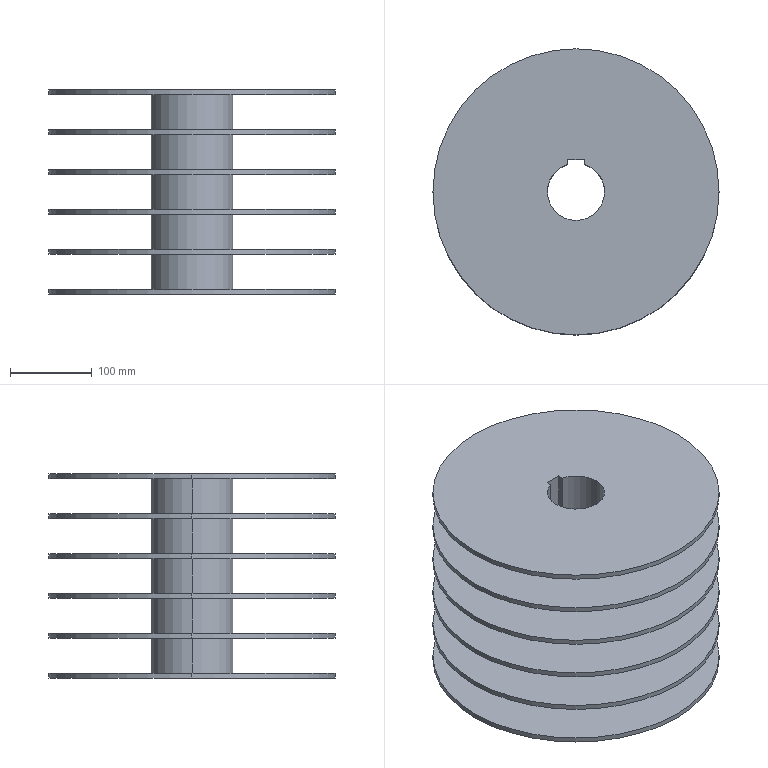Component | SolidWorks | HammerPiece-1_ToolHolder-1 | 1 solid | 40 faces | box 350 x 350 x 250 mm | volume 4155334 mm3 | cylinder 25 | plane 15 | commonest cylinder face diameters 350 x12 100 x10 70 x3
STEP:
#1=CARTESIAN_POINT('',(6.89,8.839,-4.921));
#2=VERTEX_POINT('',#1);
#3=CARTESIAN_POINT('',(9.646,8.839,-4.921));
#4=VERTEX_POINT('',#3);
#5=CARTESIAN_POINT('',(8.268,8.839,-4.921));
#6=DIRECTION('',(0.,0.,1.));
#7=DIRECTION('',(1.,0.,0.));
#8=AXIS2_PLACEMENT_3D('',#5,#6,#7);
#9=CIRCLE('',#8,1.378);
#10=EDGE_CURVE('',#2,#4,#9,.T.);
#11=ORIENTED_EDGE('',*,*,#10,.F.);
#12=CARTESIAN_POINT('',(6.89,8.839,4.921));
#13=VERTEX_POINT('',#12);
#14=CARTESIAN_POINT('',(6.89,8.839,-0.));
#15=DIRECTION('',(0.,0.,1.));
#16=VECTOR('',#15,39.37);
#17=LINE('',#14,#16);
#18=EDGE_CURVE('',#2,#13,#17,.T.);
#19=ORIENTED_EDGE('',*,*,#18,.T.);
#20=CARTESIAN_POINT('',(9.646,8.839,4.921));
#21=VERTEX_POINT('',#20);
#22=CARTESIAN_POINT('',(8.268,8.839,4.921));
#23=DIRECTION('',(0.,0.,1.));
#24=DIRECTION('',(1.,0.,0.));
#25=AXIS2_PLACEMENT_3D('',#22,#23,#24);
#26=CIRCLE('',#25,1.378);
#27=EDGE_CURVE('',#13,#21,#26,.T.);
#28=ORIENTED_EDGE('',*,*,#27,.T.);
#29=CARTESIAN_POINT('',(9.646,8.839,-0.));
#30=DIRECTION('',(0.,0.,1.));
#31=VECTOR('',#30,39.37);
#32=LINE('',#29,#31);
#33=EDGE_CURVE('',#4,#21,#32,.T.);
#34=ORIENTED_EDGE('',*,*,#33,.F.);
#35=EDGE_LOOP('',(#11,#19,#28,#34));
#36=FACE_OUTER_BOUND('',#35,.T.);
#37=CARTESIAN_POINT('',(8.268,8.839,-0.));
#38=DIRECTION('',(0.,0.,1.));
#39=DIRECTION('',(1.,0.,0.));
#40=AXIS2_PLACEMENT_3D('',#37,#38,#39);
#41=CYLINDRICAL_SURFACE('',#40,1.378);
#42=ADVANCED_FACE('',(#36),#41,.F.);
#43=CARTESIAN_POINT('',(8.661,10.159,-4.921));
#44=VERTEX_POINT('',#43);
#45=CARTESIAN_POINT('',(8.268,8.839,-4.921));
#46=DIRECTION('',(0.,0.,1.));
#47=DIRECTION('',(1.,0.,0.));
#48=AXIS2_PLACEMENT_3D('',#45,#46,#47);
#49=CIRCLE('',#48,1.378);
#50=EDGE_CURVE('',#4,#44,#49,.T.);
#51=ORIENTED_EDGE('',*,*,#50,.F.);
#52=ORIENTED_EDGE('',*,*,#33,.T.);
#53=CARTESIAN_POINT('',(8.661,10.159,4.921));
#54=VERTEX_POINT('',#53);
#55=CARTESIAN_POINT('',(8.268,8.839,4.921));
#56=DIRECTION('',(0.,0.,1.));
#57=DIRECTION('',(1.,0.,0.));
#58=AXIS2_PLACEMENT_3D('',#55,#56,#57);
#59=CIRCLE('',#58,1.378);
#60=EDGE_CURVE('',#21,#54,#59,.T.);
#61=ORIENTED_EDGE('',*,*,#60,.T.);
#62=CARTESIAN_POINT('',(8.661,10.159,5.157));
#63=DIRECTION('',(0.,0.,-1.));
#64=VECTOR('',#63,39.37);
#65=LINE('',#62,#64);
#66=EDGE_CURVE('',#54,#44,#65,.T.);
#67=ORIENTED_EDGE('',*,*,#66,.T.);
#68=EDGE_LOOP('',(#51,#52,#61,#67));
#69=FACE_OUTER_BOUND('',#68,.T.);
#70=CARTESIAN_POINT('',(8.268,8.839,-0.));
#71=DIRECTION('',(0.,0.,1.));
#72=DIRECTION('',(1.,0.,0.));
#73=AXIS2_PLACEMENT_3D('',#70,#71,#72);
#74=CYLINDRICAL_SURFACE('',#73,1.378);
#75=ADVANCED_FACE('',(#69),#74,.F.);
#76=CARTESIAN_POINT('',(15.157,8.839,4.685));
#77=VERTEX_POINT('',#76);
#78=CARTESIAN_POINT('',(1.378,8.839,4.685));
#79=VERTEX_POINT('',#78);
#80=CARTESIAN_POINT('',(8.268,8.839,4.685));
#81=DIRECTION('',(0.,0.,1.));
#82=DIRECTION('',(1.,0.,0.));
#83=AXIS2_PLACEMENT_3D('',#80,#81,#82);
#84=CIRCLE('',#83,6.89);
#85=EDGE_CURVE('',#77,#79,#84,.T.);
#86=ORIENTED_EDGE('',*,*,#85,.T.);
#87=CARTESIAN_POINT('',(1.378,8.839,4.921));
#88=VERTEX_POINT('',#87);
#89=CARTESIAN_POINT('',(1.378,8.839,-0.));
#90=DIRECTION('',(0.,0.,1.));
#91=VECTOR('',#90,39.37);
#92=LINE('',#89,#91);
#93=EDGE_CURVE('',#79,#88,#92,.T.);
#94=ORIENTED_EDGE('',*,*,#93,.T.);
#95=CARTESIAN_POINT('',(15.157,8.839,4.921));
#96=VERTEX_POINT('',#95);
#97=CARTESIAN_POINT('',(8.268,8.839,4.921));
#98=DIRECTION('',(0.,0.,-1.));
#99=DIRECTION('',(1.,0.,0.));
#100=AXIS2_PLACEMENT_3D('',#97,#98,#99);
#101=CIRCLE('',#100,6.89);
#102=EDGE_CURVE('',#88,#96,#101,.T.);
#103=ORIENTED_EDGE('',*,*,#102,.T.);
#104=CARTESIAN_POINT('',(15.157,8.839,-0.));
#105=DIRECTION('',(0.,0.,1.));
#106=VECTOR('',#105,39.37);
#107=LINE('',#104,#106);
#108=EDGE_CURVE('',#77,#96,#107,.T.);
#109=ORIENTED_EDGE('',*,*,#108,.F.);
#110=EDGE_LOOP('',(#86,#94,#103,#109));
#111=FACE_OUTER_BOUND('',#110,.T.);
#112=CARTESIAN_POINT('',(8.268,8.839,-0.));
#113=DIRECTION('',(0.,0.,1.));
#114=DIRECTION('',(1.,0.,0.));
#115=AXIS2_PLACEMENT_3D('',#112,#113,#114);
#116=CYLINDRICAL_SURFACE('',#115,6.89);
#117=ADVANCED_FACE('',(#111),#116,.T.);
#118=CARTESIAN_POINT('',(15.157,8.839,-4.921));
#119=VERTEX_POINT('',#118);
#120=CARTESIAN_POINT('',(1.378,8.839,-4.921));
#121=VERTEX_POINT('',#120);
#122=CARTESIAN_POINT('',(8.268,8.839,-4.921));
#123=DIRECTION('',(0.,0.,1.));
#124=DIRECTION('',(1.,0.,0.));
#125=AXIS2_PLACEMENT_3D('',#122,#123,#124);
#126=CIRCLE('',#125,6.89);
#127=EDGE_CURVE('',#119,#121,#126,.T.);
#128=ORIENTED_EDGE('',*,*,#127,.T.);
#129=CARTESIAN_POINT('',(1.378,8.839,-4.685));
#130=VERTEX_POINT('',#129);
#131=CARTESIAN_POINT('',(1.378,8.839,-0.));
#132=DIRECTION('',(0.,0.,1.));
#133=VECTOR('',#132,39.37);
#134=LINE('',#131,#133);
#135=EDGE_CURVE('',#121,#130,#134,.T.);
#136=ORIENTED_EDGE('',*,*,#135,.T.);
#137=CARTESIAN_POINT('',(15.157,8.839,-4.685));
#138=VERTEX_POINT('',#137);
#139=CARTESIAN_POINT('',(8.268,8.839,-4.685));
#140=DIRECTION('',(0.,0.,-1.));
#141=DIRECTION('',(1.,0.,0.));
#142=AXIS2_PLACEMENT_3D('',#139,#140,#141);
#143=CIRCLE('',#142,6.89);
#144=EDGE_CURVE('',#130,#138,#143,.T.);
#145=ORIENTED_EDGE('',*,*,#144,.T.);
#146=CARTESIAN_POINT('',(15.157,8.839,-0.));
#147=DIRECTION('',(0.,0.,1.));
#148=VECTOR('',#147,39.37);
#149=LINE('',#146,#148);
#150=EDGE_CURVE('',#119,#138,#149,.T.);
#151=ORIENTED_EDGE('',*,*,#150,.F.);
#152=EDGE_LOOP('',(#128,#136,#145,#151));
#153=FACE_OUTER_BOUND('',#152,.T.);
#154=CARTESIAN_POINT('',(8.268,8.839,-0.));
#155=DIRECTION('',(0.,0.,1.));
#156=DIRECTION('',(1.,0.,0.));
#157=AXIS2_PLACEMENT_3D('',#154,#155,#156);
#158=CYLINDRICAL_SURFACE('',#157,6.89);
#159=ADVANCED_FACE('',(#153),#158,.T.);
#160=CARTESIAN_POINT('',(10.236,8.839,3.));
#161=VERTEX_POINT('',#160);
#162=CARTESIAN_POINT('',(6.299,8.839,3.));
#163=VERTEX_POINT('',#162);
#164=CARTESIAN_POINT('',(8.268,8.839,3.));
#165=DIRECTION('',(0.,0.,1.));
#166=DIRECTION('',(1.,0.,0.));
#167=AXIS2_PLACEMENT_3D('',#164,#165,#166);
#168=CIRCLE('',#167,1.969);
#169=EDGE_CURVE('',#161,#163,#168,.T.);
#170=ORIENTED_EDGE('',*,*,#169,.T.);
#171=CARTESIAN_POINT('',(6.299,8.839,4.685));
#172=VERTEX_POINT('',#171);
#173=CARTESIAN_POINT('',(6.299,8.839,-10.489));
#174=DIRECTION('',(0.,0.,1.));
#175=VECTOR('',#174,39.37);
#176=LINE('',#173,#175);
#177=EDGE_CURVE('',#163,#172,#176,.T.);
#178=ORIENTED_EDGE('',*,*,#177,.T.);
#179=CARTESIAN_POINT('',(10.236,8.839,4.685));
#180=VERTEX_POINT('',#179);
#181=CARTESIAN_POINT('',(8.268,8.839,4.685));
#182=DIRECTION('',(0.,0.,-1.));
#183=DIRECTION('',(1.,0.,0.));
#184=AXIS2_PLACEMENT_3D('',#181,#182,#183);
#185=CIRCLE('',#184,1.969);
#186=EDGE_CURVE('',#172,#180,#185,.T.);
#187=ORIENTED_EDGE('',*,*,#186,.T.);
#188=CARTESIAN_POINT('',(10.236,8.839,-10.489));
#189=DIRECTION('',(0.,0.,1.));
#190=VECTOR('',#189,39.37);
#191=LINE('',#188,#190);
#192=EDGE_CURVE('',#161,#180,#191,.T.);
#193=ORIENTED_EDGE('',*,*,#192,.F.);
#194=EDGE_LOOP('',(#170,#178,#187,#193));
#195=FACE_OUTER_BOUND('',#194,.T.);
#196=CARTESIAN_POINT('',(8.268,8.839,-10.489));
#197=DIRECTION('',(0.,0.,1.));
#198=DIRECTION('',(1.,0.,0.));
#199=AXIS2_PLACEMENT_3D('',#196,#197,#198);
#200=CYLINDRICAL_SURFACE('',#199,1.969);
#201=ADVANCED_FACE('',(#195),#200,.T.);
#202=CARTESIAN_POINT('',(10.236,8.839,-4.685));
#203=VERTEX_POINT('',#202);
#204=CARTESIAN_POINT('',(6.299,8.839,-4.685));
#205=VERTEX_POINT('',#204);
#206=CARTESIAN_POINT('',(8.268,8.839,-4.685));
#207=DIRECTION('',(0.,0.,1.));
#208=DIRECTION('',(1.,0.,0.));
#209=AXIS2_PLACEMENT_3D('',#206,#207,#208);
#210=CIRCLE('',#209,1.969);
#211=EDGE_CURVE('',#203,#205,#210,.T.);
#212=ORIENTED_EDGE('',*,*,#211,.T.);
#213=CARTESIAN_POINT('',(6.299,8.839,-3.));
#214=VERTEX_POINT('',#213);
#215=CARTESIAN_POINT('',(6.299,8.839,-10.489));
#216=DIRECTION('',(0.,0.,1.));
#217=VECTOR('',#216,39.37);
#218=LINE('',#215,#217);
#219=EDGE_CURVE('',#205,#214,#218,.T.);
#220=ORIENTED_EDGE('',*,*,#219,.T.);
#221=CARTESIAN_POINT('',(10.236,8.839,-3.));
#222=VERTEX_POINT('',#221);
#223=CARTESIAN_POINT('',(8.268,8.839,-3.));
#224=DIRECTION('',(0.,0.,-1.));
#225=DIRECTION('',(1.,0.,0.));
#226=AXIS2_PLACEMENT_3D('',#223,#224,#225);
#227=CIRCLE('',#226,1.969);
#228=EDGE_CURVE('',#214,#222,#227,.T.);
#229=ORIENTED_EDGE('',*,*,#228,.T.);
#230=CARTESIAN_POINT('',(10.236,8.839,-10.489));
#231=DIRECTION('',(0.,0.,1.));
#232=VECTOR('',#231,39.37);
#233=LINE('',#230,#232);
#234=EDGE_CURVE('',#203,#222,#233,.T.);
#235=ORIENTED_EDGE('',*,*,#234,.F.);
#236=EDGE_LOOP('',(#212,#220,#229,#235));
#237=FACE_OUTER_BOUND('',#236,.T.);
#238=CARTESIAN_POINT('',(8.268,8.839,-10.489));
#239=DIRECTION('',(0.,0.,1.));
#240=DIRECTION('',(1.,0.,0.));
#241=AXIS2_PLACEMENT_3D('',#238,#239,#240);
#242=CYLINDRICAL_SURFACE('',#241,1.969);
#243=ADVANCED_FACE('',(#237),#242,.T.);
#244=CARTESIAN_POINT('',(15.157,8.839,2.764));
#245=VERTEX_POINT('',#244);
#246=CARTESIAN_POINT('',(1.378,8.839,2.764));
#247=VERTEX_POINT('',#246);
#248=CARTESIAN_POINT('',(8.268,8.839,2.764));
#249=DIRECTION('',(0.,0.,1.));
#250=DIRECTION('',(1.,0.,0.));
#251=AXIS2_PLACEMENT_3D('',#248,#249,#250);
#252=CIRCLE('',#251,6.89);
#253=EDGE_CURVE('',#245,#247,#252,.T.);
#254=ORIENTED_EDGE('',*,*,#253,.T.);
#255=CARTESIAN_POINT('',(1.378,8.839,3.));
#256=VERTEX_POINT('',#255);
#257=CARTESIAN_POINT('',(1.378,8.839,-0.));
#258=DIRECTION('',(0.,0.,1.));
#259=VECTOR('',#258,39.37);
#260=LINE('',#257,#259);
#261=EDGE_CURVE('',#247,#256,#260,.T.);
#262=ORIENTED_EDGE('',*,*,#261,.T.);
#263=CARTESIAN_POINT('',(15.157,8.839,3.));
#264=VERTEX_POINT('',#263);
#265=CARTESIAN_POINT('',(8.268,8.839,3.));
#266=DIRECTION('',(0.,0.,-1.));
#267=DIRECTION('',(1.,0.,0.));
#268=AXIS2_PLACEMENT_3D('',#265,#266,#267);
#269=CIRCLE('',#268,6.89);
#270=EDGE_CURVE('',#256,#264,#269,.T.);
#271=ORIENTED_EDGE('',*,*,#270,.T.);
#272=CARTESIAN_POINT('',(15.157,8.839,-0.));
#273=DIRECTION('',(0.,0.,1.));
#274=VECTOR('',#273,39.37);
#275=LINE('',#272,#274);
#276=EDGE_CURVE('',#245,#264,#275,.T.);
#277=ORIENTED_EDGE('',*,*,#276,.F.);
#278=EDGE_LOOP('',(#254,#262,#271,#277));
#279=FACE_OUTER_BOUND('',#278,.T.);
#280=CARTESIAN_POINT('',(8.268,8.839,-0.));
#281=DIRECTION('',(0.,0.,1.));
#282=DIRECTION('',(1.,0.,0.));
#283=AXIS2_PLACEMENT_3D('',#280,#281,#282);
#284=CYLINDRICAL_SURFACE('',#283,6.89);
#285=ADVANCED_FACE('',(#279),#284,.T.);
#286=CARTESIAN_POINT('',(15.157,8.839,-3.));
#287=VERTEX_POINT('',#286);
#288=CARTESIAN_POINT('',(1.378,8.839,-3.));
#289=VERTEX_POINT('',#288);
#290=CARTESIAN_POINT('',(8.268,8.839,-3.));
#291=DIRECTION('',(0.,0.,1.));
#292=DIRECTION('',(1.,0.,0.));
#293=AXIS2_PLACEMENT_3D('',#290,#291,#292);
#294=CIRCLE('',#293,6.89);
#295=EDGE_CURVE('',#287,#289,#294,.T.);
#296=ORIENTED_EDGE('',*,*,#295,.T.);
#297=CARTESIAN_POINT('',(1.378,8.839,-2.764));
#298=VERTEX_POINT('',#297);
#299=CARTESIAN_POINT('',(1.378,8.839,-0.));
#300=DIRECTION('',(0.,0.,1.));
#301=VECTOR('',#300,39.37);
#302=LINE('',#299,#301);
#303=EDGE_CURVE('',#289,#298,#302,.T.);
#304=ORIENTED_EDGE('',*,*,#303,.T.);
#305=CARTESIAN_POINT('',(15.157,8.839,-2.764));
#306=VERTEX_POINT('',#305);
#307=CARTESIAN_POINT('',(8.268,8.839,-2.764));
#308=DIRECTION('',(0.,0.,-1.));
#309=DIRECTION('',(1.,0.,0.));
#310=AXIS2_PLACEMENT_3D('',#307,#308,#309);
#311=CIRCLE('',#310,6.89);
#312=EDGE_CURVE('',#298,#306,#311,.T.);
#313=ORIENTED_EDGE('',*,*,#312,.T.);
#314=CARTESIAN_POINT('',(15.157,8.839,-0.));
#315=DIRECTION('',(0.,0.,1.));
#316=VECTOR('',#315,39.37);
#317=LINE('',#314,#316);
#318=EDGE_CURVE('',#287,#306,#317,.T.);
#319=ORIENTED_EDGE('',*,*,#318,.F.);
#320=EDGE_LOOP('',(#296,#304,#313,#319));
#321=FACE_OUTER_BOUND('',#320,.T.);
#322=CARTESIAN_POINT('',(8.268,8.839,-0.));
#323=DIRECTION('',(0.,0.,1.));
#324=DIRECTION('',(1.,0.,0.));
#325=AXIS2_PLACEMENT_3D('',#322,#323,#324);
#326=CYLINDRICAL_SURFACE('',#325,6.89);
#327=ADVANCED_FACE('',(#321),#326,.T.);
#328=CARTESIAN_POINT('',(10.236,8.839,1.079));
#329=VERTEX_POINT('',#328);
#330=CARTESIAN_POINT('',(6.299,8.839,1.079));
#331=VERTEX_POINT('',#330);
#332=CARTESIAN_POINT('',(8.268,8.839,1.079));
#333=DIRECTION('',(0.,0.,1.));
#334=DIRECTION('',(1.,0.,0.));
#335=AXIS2_PLACEMENT_3D('',#332,#333,#334);
#336=CIRCLE('',#335,1.969);
#337=EDGE_CURVE('',#329,#331,#336,.T.);
#338=ORIENTED_EDGE('',*,*,#337,.T.);
#339=CARTESIAN_POINT('',(6.299,8.839,2.764));
#340=VERTEX_POINT('',#339);
#341=CARTESIAN_POINT('',(6.299,8.839,-10.489));
#342=DIRECTION('',(0.,0.,1.));
#343=VECTOR('',#342,39.37);
#344=LINE('',#341,#343);
#345=EDGE_CURVE('',#331,#340,#344,.T.);
#346=ORIENTED_EDGE('',*,*,#345,.T.);
#347=CARTESIAN_POINT('',(10.236,8.839,2.764));
#348=VERTEX_POINT('',#347);
#349=CARTESIAN_POINT('',(8.268,8.839,2.764));
#350=DIRECTION('',(0.,0.,-1.));
#351=DIRECTION('',(1.,0.,0.));
#352=AXIS2_PLACEMENT_3D('',#349,#350,#351);
#353=CIRCLE('',#352,1.969);
#354=EDGE_CURVE('',#340,#348,#353,.T.);
#355=ORIENTED_EDGE('',*,*,#354,.T.);
#356=CARTESIAN_POINT('',(10.236,8.839,-10.489));
#357=DIRECTION('',(0.,0.,1.));
#358=VECTOR('',#357,39.37);
#359=LINE('',#356,#358);
#360=EDGE_CURVE('',#329,#348,#359,.T.);
#361=ORIENTED_EDGE('',*,*,#360,.F.);
#362=EDGE_LOOP('',(#338,#346,#355,#361));
#363=FACE_OUTER_BOUND('',#362,.T.);
#364=CARTESIAN_POINT('',(8.268,8.839,-10.489));
#365=DIRECTION('',(0.,0.,1.));
#366=DIRECTION('',(1.,0.,0.));
#367=AXIS2_PLACEMENT_3D('',#364,#365,#366);
#368=CYLINDRICAL_SURFACE('',#367,1.969);
#369=ADVANCED_FACE('',(#363),#368,.T.);
#370=CARTESIAN_POINT('',(10.236,8.839,-2.764));
#371=VERTEX_POINT('',#370);
#372=CARTESIAN_POINT('',(6.299,8.839,-2.764));
#373=VERTEX_POINT('',#372);
#374=CARTESIAN_POINT('',(8.268,8.839,-2.764));
#375=DIRECTION('',(0.,0.,1.));
#376=DIRECTION('',(1.,0.,0.));
#377=AXIS2_PLACEMENT_3D('',#374,#375,#376);
#378=CIRCLE('',#377,1.969);
#379=EDGE_CURVE('',#371,#373,#378,.T.);
#380=ORIENTED_EDGE('',*,*,#379,.T.);
#381=CARTESIAN_POINT('',(6.299,8.839,-1.079));
#382=VERTEX_POINT('',#381);
#383=CARTESIAN_POINT('',(6.299,8.839,-10.489));
#384=DIRECTION('',(0.,0.,1.));
#385=VECTOR('',#384,39.37);
#386=LINE('',#383,#385);
#387=EDGE_CURVE('',#373,#382,#386,.T.);
#388=ORIENTED_EDGE('',*,*,#387,.T.);
#389=CARTESIAN_POINT('',(10.236,8.839,-1.079));
#390=VERTEX_POINT('',#389);
#391=CARTESIAN_POINT('',(8.268,8.839,-1.079));
#392=DIRECTION('',(0.,0.,-1.));
#393=DIRECTION('',(1.,0.,0.));
#394=AXIS2_PLACEMENT_3D('',#391,#392,#393);
#395=CIRCLE('',#394,1.969);
#396=EDGE_CURVE('',#382,#390,#395,.T.);
#397=ORIENTED_EDGE('',*,*,#396,.T.);
#398=CARTESIAN_POINT('',(10.236,8.839,-10.489));
#399=DIRECTION('',(0.,0.,1.));
#400=VECTOR('',#399,39.37);
#401=LINE('',#398,#400);
#402=EDGE_CURVE('',#371,#390,#401,.T.);
#403=ORIENTED_EDGE('',*,*,#402,.F.);
#404=EDGE_LOOP('',(#380,#388,#397,#403));
#405=FACE_OUTER_BOUND('',#404,.T.);
#406=CARTESIAN_POINT('',(8.268,8.839,-10.489));
#407=DIRECTION('',(0.,0.,1.));
#408=DIRECTION('',(1.,0.,0.));
#409=AXIS2_PLACEMENT_3D('',#406,#407,#408);
#410=CYLINDRICAL_SURFACE('',#409,1.969);
#411=ADVANCED_FACE('',(#405),#410,.T.);
#412=CARTESIAN_POINT('',(15.157,8.839,0.8425));
#413=VERTEX_POINT('',#412);
#414=CARTESIAN_POINT('',(1.378,8.839,0.8425));
#415=VERTEX_POINT('',#414);
#416=CARTESIAN_POINT('',(8.268,8.839,0.8425));
#417=DIRECTION('',(0.,0.,1.));
#418=DIRECTION('',(1.,0.,0.));
#419=AXIS2_PLACEMENT_3D('',#416,#417,#418);
#420=CIRCLE('',#419,6.89);
#421=EDGE_CURVE('',#413,#415,#420,.T.);
#422=ORIENTED_EDGE('',*,*,#421,.T.);
#423=CARTESIAN_POINT('',(1.378,8.839,1.079));
#424=VERTEX_POINT('',#423);
#425=CARTESIAN_POINT('',(1.378,8.839,-0.));
#426=DIRECTION('',(0.,0.,1.));
#427=VECTOR('',#426,39.37);
#428=LINE('',#425,#427);
#429=EDGE_CURVE('',#415,#424,#428,.T.);
#430=ORIENTED_EDGE('',*,*,#429,.T.);
#431=CARTESIAN_POINT('',(15.157,8.839,1.079));
#432=VERTEX_POINT('',#431);
#433=CARTESIAN_POINT('',(8.268,8.839,1.079));
#434=DIRECTION('',(0.,0.,-1.));
#435=DIRECTION('',(1.,0.,0.));
#436=AXIS2_PLACEMENT_3D('',#433,#434,#435);
#437=CIRCLE('',#436,6.89);
#438=EDGE_CURVE('',#424,#432,#437,.T.);
#439=ORIENTED_EDGE('',*,*,#438,.T.);
#440=CARTESIAN_POINT('',(15.157,8.839,-0.));
#441=DIRECTION('',(0.,0.,1.));
#442=VECTOR('',#441,39.37);
#443=LINE('',#440,#442);
#444=EDGE_CURVE('',#413,#432,#443,.T.);
#445=ORIENTED_EDGE('',*,*,#444,.F.);
#446=EDGE_LOOP('',(#422,#430,#439,#445));
#447=FACE_OUTER_BOUND('',#446,.T.);
#448=CARTESIAN_POINT('',(8.268,8.839,-0.));
#449=DIRECTION('',(0.,0.,1.));
#450=DIRECTION('',(1.,0.,0.));
#451=AXIS2_PLACEMENT_3D('',#448,#449,#450);
#452=CYLINDRICAL_SURFACE('',#451,6.89);
#453=ADVANCED_FACE('',(#447),#452,.T.);
#454=CARTESIAN_POINT('',(15.157,8.839,-1.079));
#455=VERTEX_POINT('',#454);
#456=CARTESIAN_POINT('',(1.378,8.839,-1.079));
#457=VERTEX_POINT('',#456);
#458=CARTESIAN_POINT('',(8.268,8.839,-1.079));
#459=DIRECTION('',(0.,0.,1.));
#460=DIRECTION('',(1.,0.,0.));
#461=AXIS2_PLACEMENT_3D('',#458,#459,#460);
#462=CIRCLE('',#461,6.89);
#463=EDGE_CURVE('',#455,#457,#462,.T.);
#464=ORIENTED_EDGE('',*,*,#463,.T.);
#465=CARTESIAN_POINT('',(1.378,8.839,-0.8425));
#466=VERTEX_POINT('',#465);
#467=CARTESIAN_POINT('',(1.378,8.839,-0.));
#468=DIRECTION('',(0.,0.,1.));
#469=VECTOR('',#468,39.37);
#470=LINE('',#467,#469);
#471=EDGE_CURVE('',#457,#466,#470,.T.);
#472=ORIENTED_EDGE('',*,*,#471,.T.);
#473=CARTESIAN_POINT('',(15.157,8.839,-0.8425));
#474=VERTEX_POINT('',#473);
#475=CARTESIAN_POINT('',(8.268,8.839,-0.8425));
#476=DIRECTION('',(0.,0.,-1.));
#477=DIRECTION('',(1.,0.,0.));
#478=AXIS2_PLACEMENT_3D('',#475,#476,#477);
#479=CIRCLE('',#478,6.89);
#480=EDGE_CURVE('',#466,#474,#479,.T.);
#481=ORIENTED_EDGE('',*,*,#480,.T.);
#482=CARTESIAN_POINT('',(15.157,8.839,-0.));
#483=DIRECTION('',(0.,0.,1.));
#484=VECTOR('',#483,39.37);
#485=LINE('',#482,#484);
#486=EDGE_CURVE('',#455,#474,#485,.T.);
#487=ORIENTED_EDGE('',*,*,#486,.F.);
#488=EDGE_LOOP('',(#464,#472,#481,#487));
#489=FACE_OUTER_BOUND('',#488,.T.);
#490=CARTESIAN_POINT('',(8.268,8.839,-0.));
#491=DIRECTION('',(0.,0.,1.));
#492=DIRECTION('',(1.,0.,0.));
#493=AXIS2_PLACEMENT_3D('',#490,#491,#492);
#494=CYLINDRICAL_SURFACE('',#493,6.89);
#495=ADVANCED_FACE('',(#489),#494,.T.);
#496=CARTESIAN_POINT('',(10.236,8.839,-0.8425));
#497=VERTEX_POINT('',#496);
#498=CARTESIAN_POINT('',(6.299,8.839,-0.8425));
#499=VERTEX_POINT('',#498);
#500=CARTESIAN_POINT('',(8.268,8.839,-0.8425));
#501=DIRECTION('',(0.,0.,1.));
#502=DIRECTION('',(1.,0.,0.));
#503=AXIS2_PLACEMENT_3D('',#500,#501,#502);
#504=CIRCLE('',#503,1.969);
#505=EDGE_CURVE('',#497,#499,#504,.T.);
#506=ORIENTED_EDGE('',*,*,#505,.T.);
#507=CARTESIAN_POINT('',(6.299,8.839,0.8425));
#508=VERTEX_POINT('',#507);
#509=CARTESIAN_POINT('',(6.299,8.839,-10.489));
#510=DIRECTION('',(0.,0.,1.));
#511=VECTOR('',#510,39.37);
#512=LINE('',#509,#511);
#513=EDGE_CURVE('',#499,#508,#512,.T.);
#514=ORIENTED_EDGE('',*,*,#513,.T.);
#515=CARTESIAN_POINT('',(10.236,8.839,0.8425));
#516=VERTEX_POINT('',#515);
#517=CARTESIAN_POINT('',(8.268,8.839,0.8425));
#518=DIRECTION('',(0.,0.,-1.));
#519=DIRECTION('',(1.,0.,0.));
#520=AXIS2_PLACEMENT_3D('',#517,#518,#519);
#521=CIRCLE('',#520,1.969);
#522=EDGE_CURVE('',#508,#516,#521,.T.);
#523=ORIENTED_EDGE('',*,*,#522,.T.);
#524=CARTESIAN_POINT('',(10.236,8.839,-10.489));
#525=DIRECTION('',(0.,0.,1.));
#526=VECTOR('',#525,39.37);
#527=LINE('',#524,#526);
#528=EDGE_CURVE('',#497,#516,#527,.T.);
#529=ORIENTED_EDGE('',*,*,#528,.F.);
#530=EDGE_LOOP('',(#506,#514,#523,#529));
#531=FACE_OUTER_BOUND('',#530,.T.);
#532=CARTESIAN_POINT('',(8.268,8.839,-10.489));
#533=DIRECTION('',(0.,0.,1.));
#534=DIRECTION('',(1.,0.,0.));
#535=AXIS2_PLACEMENT_3D('',#532,#533,#534);
#536=CYLINDRICAL_SURFACE('',#535,1.969);
#537=ADVANCED_FACE('',(#531),#536,.T.);
#538=CARTESIAN_POINT('',(8.661,10.409,4.921));
#539=VERTEX_POINT('',#538);
#540=CARTESIAN_POINT('',(8.661,10.217,4.921));
#541=DIRECTION('',(0.,1.,0.));
#542=VECTOR('',#541,39.37);
#543=LINE('',#540,#542);
#544=EDGE_CURVE('',#54,#539,#543,.T.);
#545=ORIENTED_EDGE('',*,*,#544,.F.);
#546=ORIENTED_EDGE('',*,*,#60,.F.);
#547=ORIENTED_EDGE('',*,*,#27,.F.);
#548=CARTESIAN_POINT('',(7.874,10.159,4.921));
#549=VERTEX_POINT('',#548);
#550=CARTESIAN_POINT('',(8.268,8.839,4.921));
#551=DIRECTION('',(0.,0.,1.));
#552=DIRECTION('',(1.,0.,0.));
#553=AXIS2_PLACEMENT_3D('',#550,#551,#552);
#554=CIRCLE('',#553,1.378);
#555=EDGE_CURVE('',#549,#13,#554,.T.);
#556=ORIENTED_EDGE('',*,*,#555,.F.);
#557=CARTESIAN_POINT('',(7.874,10.409,4.921));
#558=VERTEX_POINT('',#557);
#559=CARTESIAN_POINT('',(7.874,10.217,4.921));
#560=DIRECTION('',(0.,-1.,0.));
#561=VECTOR('',#560,39.37);
#562=LINE('',#559,#561);
#563=EDGE_CURVE('',#558,#549,#562,.T.);
#564=ORIENTED_EDGE('',*,*,#563,.F.);
#565=CARTESIAN_POINT('',(8.268,10.409,4.921));
#566=DIRECTION('',(-1.,0.,0.));
#567=VECTOR('',#566,39.37);
#568=LINE('',#565,#567);
#569=EDGE_CURVE('',#539,#558,#568,.T.);
#570=ORIENTED_EDGE('',*,*,#569,.F.);
#571=EDGE_LOOP('',(#545,#546,#547,#556,#564,#570));
#572=FACE_BOUND('',#571,.T.);
#573=CARTESIAN_POINT('',(8.268,8.839,4.921));
#574=DIRECTION('',(0.,0.,-1.));
#575=DIRECTION('',(1.,0.,0.));
#576=AXIS2_PLACEMENT_3D('',#573,#574,#575);
#577=CIRCLE('',#576,6.89);
#578=EDGE_CURVE('',#96,#88,#577,.T.);
#579=ORIENTED_EDGE('',*,*,#578,.F.);
#580=ORIENTED_EDGE('',*,*,#102,.F.);
#581=EDGE_LOOP('',(#579,#580));
#582=FACE_OUTER_BOUND('',#581,.T.);
#583=CARTESIAN_POINT('',(8.268,10.217,4.921));
#584=DIRECTION('',(0.,0.,-1.));
#585=DIRECTION('',(-1.,0.,0.));
#586=AXIS2_PLACEMENT_3D('',#583,#584,#585);
#587=PLANE('',#586);
#588=ADVANCED_FACE('',(#572,#582),#587,.F.);
#589=CARTESIAN_POINT('',(8.661,10.409,-4.921));
#590=VERTEX_POINT('',#589);
#591=CARTESIAN_POINT('',(7.874,10.409,-4.921));
#592=VERTEX_POINT('',#591);
#593=CARTESIAN_POINT('',(8.661,10.409,-4.921));
#594=DIRECTION('',(-1.,0.,0.));
#595=VECTOR('',#594,39.37);
#596=LINE('',#593,#595);
#597=EDGE_CURVE('',#590,#592,#596,.T.);
#598=ORIENTED_EDGE('',*,*,#597,.F.);
#599=CARTESIAN_POINT('',(8.661,10.409,5.157));
#600=DIRECTION('',(0.,0.,-1.));
#601=VECTOR('',#600,39.37);
#602=LINE('',#599,#601);
#603=EDGE_CURVE('',#539,#590,#602,.T.);
#604=ORIENTED_EDGE('',*,*,#603,.F.);
#605=ORIENTED_EDGE('',*,*,#569,.T.);
#606=CARTESIAN_POINT('',(7.874,10.409,5.157));
#607=DIRECTION('',(0.,0.,1.));
#608=VECTOR('',#607,39.37);
#609=LINE('',#606,#608);
#610=EDGE_CURVE('',#592,#558,#609,.T.);
#611=ORIENTED_EDGE('',*,*,#610,.F.);
#612=EDGE_LOOP('',(#598,#604,#605,#611));
#613=FACE_OUTER_BOUND('',#612,.T.);
#614=CARTESIAN_POINT('',(8.661,10.409,5.157));
#615=DIRECTION('',(0.,1.,0.));
#616=DIRECTION('',(1.,0.,0.));
#617=AXIS2_PLACEMENT_3D('',#614,#615,#616);
#618=PLANE('',#617);
#619=ADVANCED_FACE('',(#613),#618,.F.);
#620=CARTESIAN_POINT('',(8.661,10.409,-4.921));
#621=DIRECTION('',(0.,1.,0.));
#622=VECTOR('',#621,39.37);
#623=LINE('',#620,#622);
#624=EDGE_CURVE('',#44,#590,#623,.T.);
#625=ORIENTED_EDGE('',*,*,#624,.F.);
#626=ORIENTED_EDGE('',*,*,#66,.F.);
#627=ORIENTED_EDGE('',*,*,#544,.T.);
#628=ORIENTED_EDGE('',*,*,#603,.T.);
#629=EDGE_LOOP('',(#625,#626,#627,#628));
#630=FACE_OUTER_BOUND('',#629,.T.);
#631=CARTESIAN_POINT('',(8.661,10.409,5.157));
#632=DIRECTION('',(1.,-0.,0.));
#633=DIRECTION('',(-0.,-1.,0.));
#634=AXIS2_PLACEMENT_3D('',#631,#632,#633);
#635=PLANE('',#634);
#636=ADVANCED_FACE('',(#630),#635,.F.);
#637=ORIENTED_EDGE('',*,*,#18,.F.);
#638=CARTESIAN_POINT('',(7.874,10.159,-4.921));
#639=VERTEX_POINT('',#638);
#640=CARTESIAN_POINT('',(8.268,8.839,-4.921));
#641=DIRECTION('',(0.,0.,1.));
#642=DIRECTION('',(1.,0.,0.));
#643=AXIS2_PLACEMENT_3D('',#640,#641,#642);
#644=CIRCLE('',#643,1.378);
#645=EDGE_CURVE('',#639,#2,#644,.T.);
#646=ORIENTED_EDGE('',*,*,#645,.F.);
#647=CARTESIAN_POINT('',(7.874,10.159,-0.));
#648=DIRECTION('',(0.,0.,-1.));
#649=VECTOR('',#648,39.37);
#650=LINE('',#647,#649);
#651=EDGE_CURVE('',#549,#639,#650,.T.);
#652=ORIENTED_EDGE('',*,*,#651,.F.);
#653=ORIENTED_EDGE('',*,*,#555,.T.);
#654=EDGE_LOOP('',(#637,#646,#652,#653));
#655=FACE_OUTER_BOUND('',#654,.T.);
#656=CARTESIAN_POINT('',(8.268,8.839,-0.));
#657=DIRECTION('',(0.,0.,1.));
#658=DIRECTION('',(1.,0.,0.));
#659=AXIS2_PLACEMENT_3D('',#656,#657,#658);
#660=CYLINDRICAL_SURFACE('',#659,1.378);
#661=ADVANCED_FACE('',(#655),#660,.F.);
#662=CARTESIAN_POINT('',(7.874,10.409,-4.921));
#663=DIRECTION('',(0.,-1.,0.));
#664=VECTOR('',#663,39.37);
#665=LINE('',#662,#664);
#666=EDGE_CURVE('',#592,#639,#665,.T.);
#667=ORIENTED_EDGE('',*,*,#666,.F.);
#668=ORIENTED_EDGE('',*,*,#610,.T.);
#669=ORIENTED_EDGE('',*,*,#563,.T.);
#670=ORIENTED_EDGE('',*,*,#651,.T.);
#671=EDGE_LOOP('',(#667,#668,#669,#670));
#672=FACE_OUTER_BOUND('',#671,.T.);
#673=CARTESIAN_POINT('',(7.874,10.409,5.157));
#674=DIRECTION('',(-1.,-0.,0.));
#675=DIRECTION('',(-0.,1.,0.));
#676=AXIS2_PLACEMENT_3D('',#673,#674,#675);
#677=PLANE('',#676);
#678=ADVANCED_FACE('',(#672),#677,.F.);
#679=ORIENTED_EDGE('',*,*,#93,.F.);
#680=CARTESIAN_POINT('',(8.268,8.839,4.685));
#681=DIRECTION('',(0.,0.,1.));
#682=DIRECTION('',(1.,0.,0.));
#683=AXIS2_PLACEMENT_3D('',#680,#681,#682);
#684=CIRCLE('',#683,6.89);
#685=EDGE_CURVE('',#79,#77,#684,.T.);
#686=ORIENTED_EDGE('',*,*,#685,.T.);
#687=ORIENTED_EDGE('',*,*,#108,.T.);
#688=ORIENTED_EDGE('',*,*,#578,.T.);
#689=EDGE_LOOP('',(#679,#686,#687,#688));
#690=FACE_OUTER_BOUND('',#689,.T.);
#691=CARTESIAN_POINT('',(8.268,8.839,-0.));
#692=DIRECTION('',(0.,0.,1.));
#693=DIRECTION('',(1.,0.,0.));
#694=AXIS2_PLACEMENT_3D('',#691,#692,#693);
#695=CYLINDRICAL_SURFACE('',#694,6.89);
#696=ADVANCED_FACE('',(#690),#695,.T.);
#697=ORIENTED_EDGE('',*,*,#666,.T.);
#698=ORIENTED_EDGE('',*,*,#645,.T.);
#699=ORIENTED_EDGE('',*,*,#10,.T.);
#700=ORIENTED_EDGE('',*,*,#50,.T.);
#701=ORIENTED_EDGE('',*,*,#624,.T.);
#702=ORIENTED_EDGE('',*,*,#597,.T.);
#703=EDGE_LOOP('',(#697,#698,#699,#700,#701,#702));
#704=FACE_BOUND('',#703,.T.);
#705=ORIENTED_EDGE('',*,*,#127,.F.);
#706=CARTESIAN_POINT('',(8.268,8.839,-4.921));
#707=DIRECTION('',(0.,0.,1.));
#708=DIRECTION('',(1.,0.,0.));
#709=AXIS2_PLACEMENT_3D('',#706,#707,#708);
#710=CIRCLE('',#709,6.89);
#711=EDGE_CURVE('',#121,#119,#710,.T.);
#712=ORIENTED_EDGE('',*,*,#711,.F.);
#713=EDGE_LOOP('',(#705,#712));
#714=FACE_OUTER_BOUND('',#713,.T.);
#715=CARTESIAN_POINT('',(8.268,10.217,-4.921));
#716=DIRECTION('',(0.,0.,1.));
#717=DIRECTION('',(1.,0.,0.));
#718=AXIS2_PLACEMENT_3D('',#715,#716,#717);
#719=PLANE('',#718);
#720=ADVANCED_FACE('',(#704,#714),#719,.F.);
#721=ORIENTED_EDGE('',*,*,#85,.F.);
#722=ORIENTED_EDGE('',*,*,#685,.F.);
#723=EDGE_LOOP('',(#721,#722));
#724=FACE_OUTER_BOUND('',#723,.T.);
#725=CARTESIAN_POINT('',(8.268,8.839,4.685));
#726=DIRECTION('',(0.,0.,-1.));
#727=DIRECTION('',(1.,0.,0.));
#728=AXIS2_PLACEMENT_3D('',#725,#726,#727);
#729=CIRCLE('',#728,1.969);
#730=EDGE_CURVE('',#180,#172,#729,.T.);
#731=ORIENTED_EDGE('',*,*,#730,.F.);
#732=ORIENTED_EDGE('',*,*,#186,.F.);
#733=EDGE_LOOP('',(#731,#732));
#734=FACE_BOUND('',#733,.T.);
#735=CARTESIAN_POINT('',(8.268,10.453,4.685));
#736=DIRECTION('',(0.,0.,1.));
#737=DIRECTION('',(1.,0.,0.));
#738=AXIS2_PLACEMENT_3D('',#735,#736,#737);
#739=PLANE('',#738);
#740=ADVANCED_FACE('',(#724,#734),#739,.F.);
#741=ORIENTED_EDGE('',*,*,#135,.F.);
#742=ORIENTED_EDGE('',*,*,#711,.T.);
#743=ORIENTED_EDGE('',*,*,#150,.T.);
#744=CARTESIAN_POINT('',(8.268,8.839,-4.685));
#745=DIRECTION('',(0.,0.,-1.));
#746=DIRECTION('',(1.,0.,0.));
#747=AXIS2_PLACEMENT_3D('',#744,#745,#746);
#748=CIRCLE('',#747,6.89);
#749=EDGE_CURVE('',#138,#130,#748,.T.);
#750=ORIENTED_EDGE('',*,*,#749,.T.);
#751=EDGE_LOOP('',(#741,#742,#743,#750));
#752=FACE_OUTER_BOUND('',#751,.T.);
#753=CARTESIAN_POINT('',(8.268,8.839,-0.));
#754=DIRECTION('',(0.,0.,1.));
#755=DIRECTION('',(1.,0.,0.));
#756=AXIS2_PLACEMENT_3D('',#753,#754,#755);
#757=CYLINDRICAL_SURFACE('',#756,6.89);
#758=ADVANCED_FACE('',(#752),#757,.T.);
#759=ORIENTED_EDGE('',*,*,#177,.F.);
#760=CARTESIAN_POINT('',(8.268,8.839,3.));
#761=DIRECTION('',(0.,0.,1.));
#762=DIRECTION('',(1.,0.,0.));
#763=AXIS2_PLACEMENT_3D('',#760,#761,#762);
#764=CIRCLE('',#763,1.969);
#765=EDGE_CURVE('',#163,#161,#764,.T.);
#766=ORIENTED_EDGE('',*,*,#765,.T.);
#767=ORIENTED_EDGE('',*,*,#192,.T.);
#768=ORIENTED_EDGE('',*,*,#730,.T.);
#769=EDGE_LOOP('',(#759,#766,#767,#768));
#770=FACE_OUTER_BOUND('',#769,.T.);
#771=CARTESIAN_POINT('',(8.268,8.839,-10.489));
#772=DIRECTION('',(0.,0.,1.));
#773=DIRECTION('',(1.,0.,0.));
#774=AXIS2_PLACEMENT_3D('',#771,#772,#773);
#775=CYLINDRICAL_SURFACE('',#774,1.969);
#776=ADVANCED_FACE('',(#770),#775,.T.);
#777=ORIENTED_EDGE('',*,*,#749,.F.);
#778=ORIENTED_EDGE('',*,*,#144,.F.);
#779=EDGE_LOOP('',(#777,#778));
#780=FACE_OUTER_BOUND('',#779,.T.);
#781=ORIENTED_EDGE('',*,*,#211,.F.);
#782=CARTESIAN_POINT('',(8.268,8.839,-4.685));
#783=DIRECTION('',(0.,0.,1.));
#784=DIRECTION('',(1.,0.,0.));
#785=AXIS2_PLACEMENT_3D('',#782,#783,#784);
#786=CIRCLE('',#785,1.969);
#787=EDGE_CURVE('',#205,#203,#786,.T.);
#788=ORIENTED_EDGE('',*,*,#787,.F.);
#789=EDGE_LOOP('',(#781,#788));
#790=FACE_BOUND('',#789,.T.);
#791=CARTESIAN_POINT('',(8.268,10.453,-4.685));
#792=DIRECTION('',(0.,0.,-1.));
#793=DIRECTION('',(-1.,0.,0.));
#794=AXIS2_PLACEMENT_3D('',#791,#792,#793);
#795=PLANE('',#794);
#796=ADVANCED_FACE('',(#780,#790),#795,.F.);
#797=CARTESIAN_POINT('',(8.268,8.839,3.));
#798=DIRECTION('',(0.,0.,-1.));
#799=DIRECTION('',(1.,0.,0.));
#800=AXIS2_PLACEMENT_3D('',#797,#798,#799);
#801=CIRCLE('',#800,6.89);
#802=EDGE_CURVE('',#264,#256,#801,.T.);
#803=ORIENTED_EDGE('',*,*,#802,.F.);
#804=ORIENTED_EDGE('',*,*,#270,.F.);
#805=EDGE_LOOP('',(#803,#804));
#806=FACE_OUTER_BOUND('',#805,.T.);
#807=ORIENTED_EDGE('',*,*,#169,.F.);
#808=ORIENTED_EDGE('',*,*,#765,.F.);
#809=EDGE_LOOP('',(#807,#808));
#810=FACE_BOUND('',#809,.T.);
#811=CARTESIAN_POINT('',(8.268,15.728,3.));
#812=DIRECTION('',(0.,0.,-1.));
#813=DIRECTION('',(-1.,0.,0.));
#814=AXIS2_PLACEMENT_3D('',#811,#812,#813);
#815=PLANE('',#814);
#816=ADVANCED_FACE('',(#806,#810),#815,.F.);
#817=ORIENTED_EDGE('',*,*,#219,.F.);
#818=ORIENTED_EDGE('',*,*,#787,.T.);
#819=ORIENTED_EDGE('',*,*,#234,.T.);
#820=CARTESIAN_POINT('',(8.268,8.839,-3.));
#821=DIRECTION('',(0.,0.,-1.));
#822=DIRECTION('',(1.,0.,0.));
#823=AXIS2_PLACEMENT_3D('',#820,#821,#822);
#824=CIRCLE('',#823,1.969);
#825=EDGE_CURVE('',#222,#214,#824,.T.);
#826=ORIENTED_EDGE('',*,*,#825,.T.);
#827=EDGE_LOOP('',(#817,#818,#819,#826));
#828=FACE_OUTER_BOUND('',#827,.T.);
#829=CARTESIAN_POINT('',(8.268,8.839,-10.489));
#830=DIRECTION('',(0.,0.,1.));
#831=DIRECTION('',(1.,0.,0.));
#832=AXIS2_PLACEMENT_3D('',#829,#830,#831);
#833=CYLINDRICAL_SURFACE('',#832,1.969);
#834=ADVANCED_FACE('',(#828),#833,.T.);
#835=ORIENTED_EDGE('',*,*,#261,.F.);
#836=CARTESIAN_POINT('',(8.268,8.839,2.764));
#837=DIRECTION('',(0.,0.,1.));
#838=DIRECTION('',(1.,0.,0.));
#839=AXIS2_PLACEMENT_3D('',#836,#837,#838);
#840=CIRCLE('',#839,6.89);
#841=EDGE_CURVE('',#247,#245,#840,.T.);
#842=ORIENTED_EDGE('',*,*,#841,.T.);
#843=ORIENTED_EDGE('',*,*,#276,.T.);
#844=ORIENTED_EDGE('',*,*,#802,.T.);
#845=EDGE_LOOP('',(#835,#842,#843,#844));
#846=FACE_OUTER_BOUND('',#845,.T.);
#847=CARTESIAN_POINT('',(8.268,8.839,-0.));
#848=DIRECTION('',(0.,0.,1.));
#849=DIRECTION('',(1.,0.,0.));
#850=AXIS2_PLACEMENT_3D('',#847,#848,#849);
#851=CYLINDRICAL_SURFACE('',#850,6.89);
#852=ADVANCED_FACE('',(#846),#851,.T.);
#853=ORIENTED_EDGE('',*,*,#295,.F.);
#854=CARTESIAN_POINT('',(8.268,8.839,-3.));
#855=DIRECTION('',(0.,0.,1.));
#856=DIRECTION('',(1.,0.,0.));
#857=AXIS2_PLACEMENT_3D('',#854,#855,#856);
#858=CIRCLE('',#857,6.89);
#859=EDGE_CURVE('',#289,#287,#858,.T.);
#860=ORIENTED_EDGE('',*,*,#859,.F.);
#861=EDGE_LOOP('',(#853,#860));
#862=FACE_OUTER_BOUND('',#861,.T.);
#863=ORIENTED_EDGE('',*,*,#825,.F.);
#864=ORIENTED_EDGE('',*,*,#228,.F.);
#865=EDGE_LOOP('',(#863,#864));
#866=FACE_BOUND('',#865,.T.);
#867=CARTESIAN_POINT('',(8.268,15.728,-3.));
#868=DIRECTION('',(0.,0.,1.));
#869=DIRECTION('',(1.,0.,0.));
#870=AXIS2_PLACEMENT_3D('',#867,#868,#869);
#871=PLANE('',#870);
#872=ADVANCED_FACE('',(#862,#866),#871,.F.);
#873=ORIENTED_EDGE('',*,*,#253,.F.);
#874=ORIENTED_EDGE('',*,*,#841,.F.);
#875=EDGE_LOOP('',(#873,#874));
#876=FACE_OUTER_BOUND('',#875,.T.);
#877=CARTESIAN_POINT('',(8.268,8.839,2.764));
#878=DIRECTION('',(0.,0.,-1.));
#879=DIRECTION('',(1.,0.,0.));
#880=AXIS2_PLACEMENT_3D('',#877,#878,#879);
#881=CIRCLE('',#880,1.969);
#882=EDGE_CURVE('',#348,#340,#881,.T.);
#883=ORIENTED_EDGE('',*,*,#882,.F.);
#884=ORIENTED_EDGE('',*,*,#354,.F.);
#885=EDGE_LOOP('',(#883,#884));
#886=FACE_BOUND('',#885,.T.);
#887=CARTESIAN_POINT('',(8.268,15.728,2.764));
#888=DIRECTION('',(0.,0.,1.));
#889=DIRECTION('',(1.,0.,0.));
#890=AXIS2_PLACEMENT_3D('',#887,#888,#889);
#891=PLANE('',#890);
#892=ADVANCED_FACE('',(#876,#886),#891,.F.);
#893=ORIENTED_EDGE('',*,*,#303,.F.);
#894=ORIENTED_EDGE('',*,*,#859,.T.);
#895=ORIENTED_EDGE('',*,*,#318,.T.);
#896=CARTESIAN_POINT('',(8.268,8.839,-2.764));
#897=DIRECTION('',(0.,0.,-1.));
#898=DIRECTION('',(1.,0.,0.));
#899=AXIS2_PLACEMENT_3D('',#896,#897,#898);
#900=CIRCLE('',#899,6.89);
#901=EDGE_CURVE('',#306,#298,#900,.T.);
#902=ORIENTED_EDGE('',*,*,#901,.T.);
#903=EDGE_LOOP('',(#893,#894,#895,#902));
#904=FACE_OUTER_BOUND('',#903,.T.);
#905=CARTESIAN_POINT('',(8.268,8.839,-0.));
#906=DIRECTION('',(0.,0.,1.));
#907=DIRECTION('',(1.,0.,0.));
#908=AXIS2_PLACEMENT_3D('',#905,#906,#907);
#909=CYLINDRICAL_SURFACE('',#908,6.89);
#910=ADVANCED_FACE('',(#904),#909,.T.);
#911=ORIENTED_EDGE('',*,*,#345,.F.);
#912=CARTESIAN_POINT('',(8.268,8.839,1.079));
#913=DIRECTION('',(0.,0.,1.));
#914=DIRECTION('',(1.,0.,0.));
#915=AXIS2_PLACEMENT_3D('',#912,#913,#914);
#916=CIRCLE('',#915,1.969);
#917=EDGE_CURVE('',#331,#329,#916,.T.);
#918=ORIENTED_EDGE('',*,*,#917,.T.);
#919=ORIENTED_EDGE('',*,*,#360,.T.);
#920=ORIENTED_EDGE('',*,*,#882,.T.);
#921=EDGE_LOOP('',(#911,#918,#919,#920));
#922=FACE_OUTER_BOUND('',#921,.T.);
#923=CARTESIAN_POINT('',(8.268,8.839,-10.489));
#924=DIRECTION('',(0.,0.,1.));
#925=DIRECTION('',(1.,0.,0.));
#926=AXIS2_PLACEMENT_3D('',#923,#924,#925);
#927=CYLINDRICAL_SURFACE('',#926,1.969);
#928=ADVANCED_FACE('',(#922),#927,.T.);
#929=ORIENTED_EDGE('',*,*,#901,.F.);
#930=ORIENTED_EDGE('',*,*,#312,.F.);
#931=EDGE_LOOP('',(#929,#930));
#932=FACE_OUTER_BOUND('',#931,.T.);
#933=ORIENTED_EDGE('',*,*,#379,.F.);
#934=CARTESIAN_POINT('',(8.268,8.839,-2.764));
#935=DIRECTION('',(0.,0.,1.));
#936=DIRECTION('',(1.,0.,0.));
#937=AXIS2_PLACEMENT_3D('',#934,#935,#936);
#938=CIRCLE('',#937,1.969);
#939=EDGE_CURVE('',#373,#371,#938,.T.);
#940=ORIENTED_EDGE('',*,*,#939,.F.);
#941=EDGE_LOOP('',(#933,#940));
#942=FACE_BOUND('',#941,.T.);
#943=CARTESIAN_POINT('',(8.268,15.728,-2.764));
#944=DIRECTION('',(0.,0.,-1.));
#945=DIRECTION('',(-1.,0.,0.));
#946=AXIS2_PLACEMENT_3D('',#943,#944,#945);
#947=PLANE('',#946);
#948=ADVANCED_FACE('',(#932,#942),#947,.F.);
#949=CARTESIAN_POINT('',(8.268,8.839,1.079));
#950=DIRECTION('',(0.,0.,-1.));
#951=DIRECTION('',(1.,0.,0.));
#952=AXIS2_PLACEMENT_3D('',#949,#950,#951);
#953=CIRCLE('',#952,6.89);
#954=EDGE_CURVE('',#432,#424,#953,.T.);
#955=ORIENTED_EDGE('',*,*,#954,.F.);
#956=ORIENTED_EDGE('',*,*,#438,.F.);
#957=EDGE_LOOP('',(#955,#956));
#958=FACE_OUTER_BOUND('',#957,.T.);
#959=ORIENTED_EDGE('',*,*,#337,.F.);
#960=ORIENTED_EDGE('',*,*,#917,.F.);
#961=EDGE_LOOP('',(#959,#960));
#962=FACE_BOUND('',#961,.T.);
#963=CARTESIAN_POINT('',(8.268,15.728,1.079));
#964=DIRECTION('',(0.,0.,-1.));
#965=DIRECTION('',(-1.,0.,0.));
#966=AXIS2_PLACEMENT_3D('',#963,#964,#965);
#967=PLANE('',#966);
#968=ADVANCED_FACE('',(#958,#962),#967,.F.);
#969=ORIENTED_EDGE('',*,*,#387,.F.);
#970=ORIENTED_EDGE('',*,*,#939,.T.);
#971=ORIENTED_EDGE('',*,*,#402,.T.);
#972=CARTESIAN_POINT('',(8.268,8.839,-1.079));
#973=DIRECTION('',(0.,0.,-1.));
#974=DIRECTION('',(1.,0.,0.));
#975=AXIS2_PLACEMENT_3D('',#972,#973,#974);
#976=CIRCLE('',#975,1.969);
#977=EDGE_CURVE('',#390,#382,#976,.T.);
#978=ORIENTED_EDGE('',*,*,#977,.T.);
#979=EDGE_LOOP('',(#969,#970,#971,#978));
#980=FACE_OUTER_BOUND('',#979,.T.);
#981=CARTESIAN_POINT('',(8.268,8.839,-10.489));
#982=DIRECTION('',(0.,0.,1.));
#983=DIRECTION('',(1.,0.,0.));
#984=AXIS2_PLACEMENT_3D('',#981,#982,#983);
#985=CYLINDRICAL_SURFACE('',#984,1.969);
#986=ADVANCED_FACE('',(#980),#985,.T.);
#987=ORIENTED_EDGE('',*,*,#429,.F.);
#988=CARTESIAN_POINT('',(8.268,8.839,0.8425));
#989=DIRECTION('',(0.,0.,1.));
#990=DIRECTION('',(1.,0.,0.));
#991=AXIS2_PLACEMENT_3D('',#988,#989,#990);
#992=CIRCLE('',#991,6.89);
#993=EDGE_CURVE('',#415,#413,#992,.T.);
#994=ORIENTED_EDGE('',*,*,#993,.T.);
#995=ORIENTED_EDGE('',*,*,#444,.T.);
#996=ORIENTED_EDGE('',*,*,#954,.T.);
#997=EDGE_LOOP('',(#987,#994,#995,#996));
#998=FACE_OUTER_BOUND('',#997,.T.);
#999=CARTESIAN_POINT('',(8.268,8.839,-0.));
#1000=DIRECTION('',(0.,0.,1.));
#1001=DIRECTION('',(1.,0.,0.));
#1002=AXIS2_PLACEMENT_3D('',#999,#1000,#1001);
#1003=CYLINDRICAL_SURFACE('',#1002,6.89);
#1004=ADVANCED_FACE('',(#998),#1003,.T.);
#1005=ORIENTED_EDGE('',*,*,#463,.F.);
#1006=CARTESIAN_POINT('',(8.268,8.839,-1.079));
#1007=DIRECTION('',(0.,0.,1.));
#1008=DIRECTION('',(1.,0.,0.));
#1009=AXIS2_PLACEMENT_3D('',#1006,#1007,#1008);
#1010=CIRCLE('',#1009,6.89);
#1011=EDGE_CURVE('',#457,#455,#1010,.T.);
#1012=ORIENTED_EDGE('',*,*,#1011,.F.);
#1013=EDGE_LOOP('',(#1005,#1012));
#1014=FACE_OUTER_BOUND('',#1013,.T.);
#1015=ORIENTED_EDGE('',*,*,#977,.F.);
#1016=ORIENTED_EDGE('',*,*,#396,.F.);
#1017=EDGE_LOOP('',(#1015,#1016));
#1018=FACE_BOUND('',#1017,.T.);
#1019=CARTESIAN_POINT('',(8.268,15.728,-1.079));
#1020=DIRECTION('',(0.,0.,1.));
#1021=DIRECTION('',(1.,0.,0.));
#1022=AXIS2_PLACEMENT_3D('',#1019,#1020,#1021);
#1023=PLANE('',#1022);
#1024=ADVANCED_FACE('',(#1014,#1018),#1023,.F.);
#1025=ORIENTED_EDGE('',*,*,#421,.F.);
#1026=ORIENTED_EDGE('',*,*,#993,.F.);
#1027=EDGE_LOOP('',(#1025,#1026));
#1028=FACE_OUTER_BOUND('',#1027,.T.);
#1029=CARTESIAN_POINT('',(8.268,8.839,0.8425));
#1030=DIRECTION('',(0.,0.,-1.));
#1031=DIRECTION('',(1.,0.,0.));
#1032=AXIS2_PLACEMENT_3D('',#1029,#1030,#1031);
#1033=CIRCLE('',#1032,1.969);
#1034=EDGE_CURVE('',#516,#508,#1033,.T.);
#1035=ORIENTED_EDGE('',*,*,#1034,.F.);
#1036=ORIENTED_EDGE('',*,*,#522,.F.);
#1037=EDGE_LOOP('',(#1035,#1036));
#1038=FACE_BOUND('',#1037,.T.);
#1039=CARTESIAN_POINT('',(8.268,15.728,0.8425));
#1040=DIRECTION('',(0.,0.,1.));
#1041=DIRECTION('',(1.,0.,0.));
#1042=AXIS2_PLACEMENT_3D('',#1039,#1040,#1041);
#1043=PLANE('',#1042);
#1044=ADVANCED_FACE('',(#1028,#1038),#1043,.F.);
#1045=ORIENTED_EDGE('',*,*,#471,.F.);
#1046=ORIENTED_EDGE('',*,*,#1011,.T.);
#1047=ORIENTED_EDGE('',*,*,#486,.T.);
#1048=CARTESIAN_POINT('',(8.268,8.839,-0.8425));
#1049=DIRECTION('',(0.,0.,-1.));
#1050=DIRECTION('',(1.,0.,0.));
#1051=AXIS2_PLACEMENT_3D('',#1048,#1049,#1050);
#1052=CIRCLE('',#1051,6.89);
#1053=EDGE_CURVE('',#474,#466,#1052,.T.);
#1054=ORIENTED_EDGE('',*,*,#1053,.T.);
#1055=EDGE_LOOP('',(#1045,#1046,#1047,#1054));
#1056=FACE_OUTER_BOUND('',#1055,.T.);
#1057=CARTESIAN_POINT('',(8.268,8.839,-0.));
#1058=DIRECTION('',(0.,0.,1.));
#1059=DIRECTION('',(1.,0.,0.));
#1060=AXIS2_PLACEMENT_3D('',#1057,#1058,#1059);
#1061=CYLINDRICAL_SURFACE('',#1060,6.89);
#1062=ADVANCED_FACE('',(#1056),#1061,.T.);
#1063=ORIENTED_EDGE('',*,*,#513,.F.);
#1064=CARTESIAN_POINT('',(8.268,8.839,-0.8425));
#1065=DIRECTION('',(0.,0.,1.));
#1066=DIRECTION('',(1.,0.,0.));
#1067=AXIS2_PLACEMENT_3D('',#1064,#1065,#1066);
#1068=CIRCLE('',#1067,1.969);
#1069=EDGE_CURVE('',#499,#497,#1068,.T.);
#1070=ORIENTED_EDGE('',*,*,#1069,.T.);
#1071=ORIENTED_EDGE('',*,*,#528,.T.);
#1072=ORIENTED_EDGE('',*,*,#1034,.T.);
#1073=EDGE_LOOP('',(#1063,#1070,#1071,#1072));
#1074=FACE_OUTER_BOUND('',#1073,.T.);
#1075=CARTESIAN_POINT('',(8.268,8.839,-10.489));
#1076=DIRECTION('',(0.,0.,1.));
#1077=DIRECTION('',(1.,0.,0.));
#1078=AXIS2_PLACEMENT_3D('',#1075,#1076,#1077);
#1079=CYLINDRICAL_SURFACE('',#1078,1.969);
#1080=ADVANCED_FACE('',(#1074),#1079,.T.);
#1081=ORIENTED_EDGE('',*,*,#1053,.F.);
#1082=ORIENTED_EDGE('',*,*,#480,.F.);
#1083=EDGE_LOOP('',(#1081,#1082));
#1084=FACE_OUTER_BOUND('',#1083,.T.);
#1085=ORIENTED_EDGE('',*,*,#505,.F.);
#1086=ORIENTED_EDGE('',*,*,#1069,.F.);
#1087=EDGE_LOOP('',(#1085,#1086));
#1088=FACE_BOUND('',#1087,.T.);
#1089=CARTESIAN_POINT('',(8.268,15.728,-0.8425));
#1090=DIRECTION('',(0.,0.,-1.));
#1091=DIRECTION('',(-1.,0.,0.));
#1092=AXIS2_PLACEMENT_3D('',#1089,#1090,#1091);
#1093=PLANE('',#1092);
#1094=ADVANCED_FACE('',(#1084,#1088),#1093,.F.);
#1095=CLOSED_SHELL('',(#42,#75,#117,#159,#201,#243,#285,#327,#369,#411,#453,#495,#537,#588,#619,#636,#661,#678,#696,#720,#740,#758,#776,#796,#816,#834,#852,#872,#892,#910,#928,#948,#968,#986,#1004,#1024,#1044,#1062,#1080,#1094));
#1096=MANIFOLD_SOLID_BREP('',#1095);
#1097=CARTESIAN_POINT('',(0.,0.,0.));
#1098=DIRECTION('',(0.,0.,1.));
#1099=DIRECTION('',(1.,0.,0.));
#1100=AXIS2_PLACEMENT_3D('',#1097,#1098,#1099);
#1101=(LENGTH_UNIT()NAMED_UNIT(*)SI_UNIT($,.METRE.));
#1102=LENGTH_MEASURE_WITH_UNIT(LENGTH_MEASURE(0.0254),#1101);
#1103=DIMENSIONAL_EXPONENTS(1.,0.,0.,0.,0.,0.,0.);
#1104=(CONVERSION_BASED_UNIT('',#1102)LENGTH_UNIT()NAMED_UNIT(#1103));
#1105=UNCERTAINTY_MEASURE_WITH_UNIT(LENGTH_MEASURE(0.00001),#1104,'','');
#1106=(NAMED_UNIT(*)PLANE_ANGLE_UNIT()SI_UNIT($,.RADIAN.));
#1107=(NAMED_UNIT(*)SI_UNIT($,.STERADIAN.)SOLID_ANGLE_UNIT());
#1108=(GEOMETRIC_REPRESENTATION_CONTEXT(3)GLOBAL_UNCERTAINTY_ASSIGNED_CONTEXT((#1105))GLOBAL_UNIT_ASSIGNED_CONTEXT((#1104,#1106,#1107))REPRESENTATION_CONTEXT('',''));
#1109=ADVANCED_BREP_SHAPE_REPRESENTATION('',(#1096,#1100),#1108);
#1110=COLOUR_RGB('',0.7922,0.8196,0.9333);
#1111=FILL_AREA_STYLE_COLOUR('',#1110);
#1112=FILL_AREA_STYLE('',(#1111));
#1113=SURFACE_STYLE_FILL_AREA(#1112);
#1114=SURFACE_SIDE_STYLE('',(#1113));
#1115=SURFACE_STYLE_USAGE(.BOTH.,#1114);
#1116=PRESENTATION_STYLE_ASSIGNMENT((#1115));
#1117=STYLED_ITEM('',(#1116),#1096);
#1118=PRESENTATION_LAYER_ASSIGNMENT('','',(#1117));
#1119=(LENGTH_UNIT()NAMED_UNIT(*)SI_UNIT($,.METRE.));
#1120=LENGTH_MEASURE_WITH_UNIT(LENGTH_MEASURE(0.0254),#1119);
#1121=DIMENSIONAL_EXPONENTS(1.,0.,0.,0.,0.,0.,0.);
#1122=(CONVERSION_BASED_UNIT('',#1120)LENGTH_UNIT()NAMED_UNIT(#1121));
#1123=UNCERTAINTY_MEASURE_WITH_UNIT(LENGTH_MEASURE(0.00001),#1122,'','');
#1124=(NAMED_UNIT(*)PLANE_ANGLE_UNIT()SI_UNIT($,.RADIAN.));
#1125=(NAMED_UNIT(*)SI_UNIT($,.STERADIAN.)SOLID_ANGLE_UNIT());
#1126=(GEOMETRIC_REPRESENTATION_CONTEXT(3)GLOBAL_UNCERTAINTY_ASSIGNED_CONTEXT((#1123))GLOBAL_UNIT_ASSIGNED_CONTEXT((#1122,#1124,#1125))REPRESENTATION_CONTEXT('',''));
#1127=MECHANICAL_DESIGN_GEOMETRIC_PRESENTATION_REPRESENTATION('',(#1117),#1126);